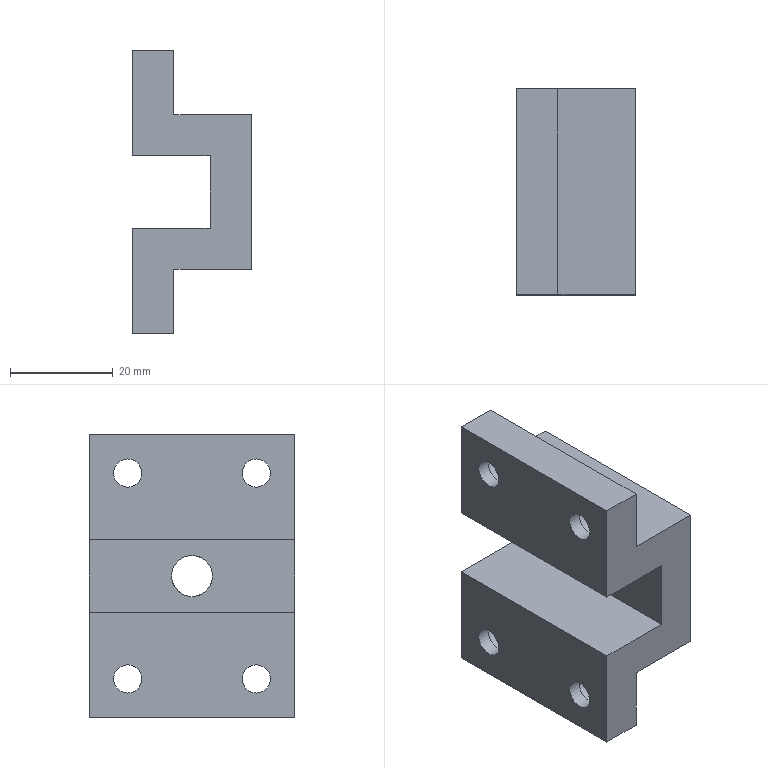Component | NX | CLAMP_SUPPORT | 1 solid | 27 faces | volume 24854 mm3 | plane 18 | cylinder 9 | commonest cylinder face diameters 5.5 x4 10 x4 8 x1